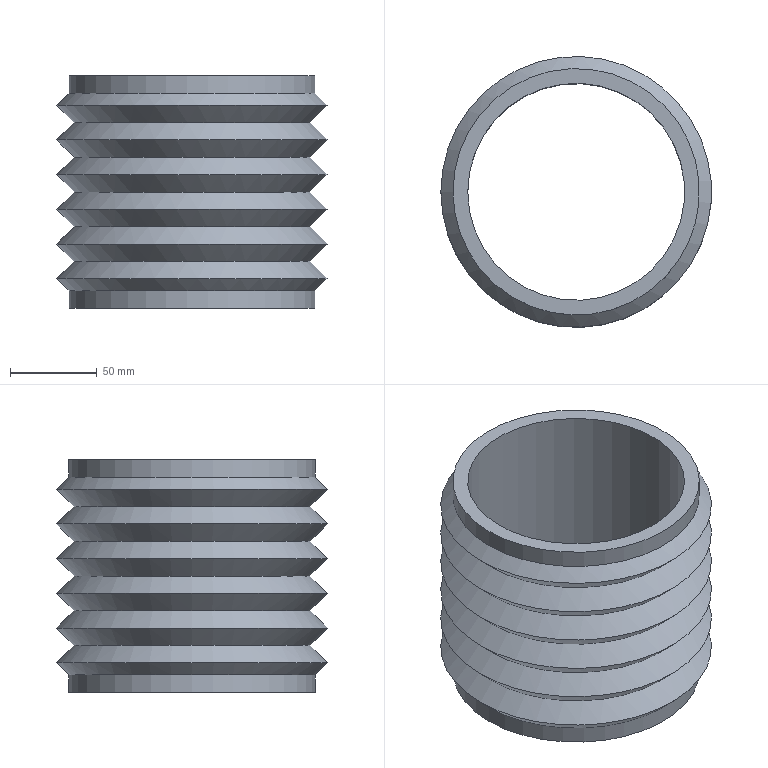Component | NX | CH3404_9-2 | 1 solid | 17 faces | box 156 x 156 x 134 mm | volume 593373 mm3 | cone 12 | cylinder 3 | plane 2 | commonest cylinder face diameters 142 x2 125 x1
STEP:
#1=CARTESIAN_POINT('',(0.,0.,0.));
#2=DIRECTION('',(0.,0.,1.));
#3=DIRECTION('',(1.,0.,0.));
#4=AXIS2_PLACEMENT_3D('',#1,#2,#3);
#5=CARTESIAN_POINT('',(-62.5,0.,0.));
#6=VERTEX_POINT('',#5);
#7=CARTESIAN_POINT('',(0.,0.,0.));
#8=DIRECTION('',(0.,0.,-1.));
#9=DIRECTION('',(-1.,0.,0.));
#10=AXIS2_PLACEMENT_3D('',#7,#8,#9);
#11=CIRCLE('',#10,62.5);
#12=CARTESIAN_POINT('',(0.,0.,-134.));
#13=DIRECTION('',(0.,0.,-1.));
#14=DIRECTION('',(-1.,0.,0.));
#15=AXIS2_PLACEMENT_3D('',#12,#13,#14);
#16=CYLINDRICAL_SURFACE('',#15,62.5);
#17=CARTESIAN_POINT('',(0.,-134.));
#18=DIRECTION('',(1.,0.));
#19=VECTOR('',#18,1.);
#20=LINE('',#17,#19);
#21=(GEOMETRIC_REPRESENTATION_CONTEXT(2)PARAMETRIC_REPRESENTATION_CONTEXT()REPRESENTATION_CONTEXT('',''));
#22=DEFINITIONAL_REPRESENTATION('',(#20),#21);
#23=PCURVE('',#16,#22);
#24=CARTESIAN_POINT('',(-62.5,0.,0.));
#25=DIRECTION('',(0.,0.,-1.));
#26=DIRECTION('',(-1.,0.,0.));
#27=AXIS2_PLACEMENT_3D('',#24,#25,#26);
#28=PLANE('',#27);
#29=CARTESIAN_POINT('',(-62.5,0.));
#30=DIRECTION('',(1.,0.));
#31=AXIS2_PLACEMENT_2D('',#29,#30);
#32=CIRCLE('',#31,62.5);
#33=(GEOMETRIC_REPRESENTATION_CONTEXT(2)PARAMETRIC_REPRESENTATION_CONTEXT()REPRESENTATION_CONTEXT('',''));
#34=DEFINITIONAL_REPRESENTATION('',(#32),#33);
#35=PCURVE('',#28,#34);
#36=SURFACE_CURVE('',#11,(#23,#35),.PCURVE_S1.);
#37=EDGE_CURVE('',#6,#6,#36,.T.);
#38=ORIENTED_EDGE('',*,*,#37,.T.);
#39=CARTESIAN_POINT('',(-62.5,0.,-134.));
#40=VERTEX_POINT('',#39);
#41=CARTESIAN_POINT('',(-62.5,0.,0.));
#42=CARTESIAN_POINT('',(-62.5,0.,-134.));
#43=B_SPLINE_CURVE_WITH_KNOTS('',1,(#41,#42),.UNSPECIFIED.,.F.,.F.,(2,2),(-134.,0.),.PIECEWISE_BEZIER_KNOTS.);
#44=CARTESIAN_POINT('',(6.283,0.));
#45=DIRECTION('',(0.,1.));
#46=VECTOR('',#45,1.);
#47=LINE('',#44,#46);
#48=(GEOMETRIC_REPRESENTATION_CONTEXT(2)PARAMETRIC_REPRESENTATION_CONTEXT()REPRESENTATION_CONTEXT('',''));
#49=DEFINITIONAL_REPRESENTATION('',(#47),#48);
#50=PCURVE('',#16,#49);
#51=CARTESIAN_POINT('',(0.,0.));
#52=DIRECTION('',(0.,1.));
#53=VECTOR('',#52,1.);
#54=LINE('',#51,#53);
#55=(GEOMETRIC_REPRESENTATION_CONTEXT(2)PARAMETRIC_REPRESENTATION_CONTEXT()REPRESENTATION_CONTEXT('',''));
#56=DEFINITIONAL_REPRESENTATION('',(#54),#55);
#57=PCURVE('',#16,#56);
#58=SEAM_CURVE('',#43,(#50,#57),.PCURVE_S1.);
#59=EDGE_CURVE('',#6,#40,#58,.T.);
#60=ORIENTED_EDGE('',*,*,#59,.T.);
#61=CARTESIAN_POINT('',(0.,0.,-134.));
#62=DIRECTION('',(0.,0.,-1.));
#63=DIRECTION('',(-1.,0.,0.));
#64=AXIS2_PLACEMENT_3D('',#61,#62,#63);
#65=CIRCLE('',#64,62.5);
#66=CARTESIAN_POINT('',(0.,0.));
#67=DIRECTION('',(1.,0.));
#68=VECTOR('',#67,1.);
#69=LINE('',#66,#68);
#70=(GEOMETRIC_REPRESENTATION_CONTEXT(2)PARAMETRIC_REPRESENTATION_CONTEXT()REPRESENTATION_CONTEXT('',''));
#71=DEFINITIONAL_REPRESENTATION('',(#69),#70);
#72=PCURVE('',#16,#71);
#73=CARTESIAN_POINT('',(-71.,0.,-134.));
#74=DIRECTION('',(0.,0.,1.));
#75=DIRECTION('',(1.,0.,0.));
#76=AXIS2_PLACEMENT_3D('',#73,#74,#75);
#77=PLANE('',#76);
#78=CARTESIAN_POINT('',(8.5,0.));
#79=CARTESIAN_POINT('',(8.5,108.253));
#80=CARTESIAN_POINT('',(102.25,54.127));
#81=CARTESIAN_POINT('',(196.,0.));
#82=CARTESIAN_POINT('',(102.25,-54.127));
#83=CARTESIAN_POINT('',(8.5,-108.253));
#84=CARTESIAN_POINT('',(8.5,0.));
#85=(BOUNDED_CURVE()B_SPLINE_CURVE(2,(#78,#79,#80,#81,#82,#83,#84),.UNSPECIFIED.,.T.,.F.)B_SPLINE_CURVE_WITH_KNOTS((1,2,2,2,2,1),(-2.094,0.,2.094,4.189,6.283,8.378),.UNSPECIFIED.)CURVE()GEOMETRIC_REPRESENTATION_ITEM()RATIONAL_B_SPLINE_CURVE((1.,0.5,1.,0.5,1.,0.5,1.))REPRESENTATION_ITEM(''));
#86=(GEOMETRIC_REPRESENTATION_CONTEXT(2)PARAMETRIC_REPRESENTATION_CONTEXT()REPRESENTATION_CONTEXT('',''));
#87=DEFINITIONAL_REPRESENTATION('',(#85),#86);
#88=PCURVE('',#77,#87);
#89=SURFACE_CURVE('',#65,(#72,#88),.PCURVE_S1.);
#90=EDGE_CURVE('',#40,#40,#89,.T.);
#91=ORIENTED_EDGE('',*,*,#90,.F.);
#92=ORIENTED_EDGE('',*,*,#59,.F.);
#93=EDGE_LOOP('',(#38,#60,#91,#92));
#94=FACE_BOUND('',#93,.F.);
#95=ADVANCED_FACE('',(#94),#16,.F.);
#96=CARTESIAN_POINT('',(-71.,0.,-0.));
#97=VERTEX_POINT('',#96);
#98=CARTESIAN_POINT('',(0.,0.,-0.));
#99=DIRECTION('',(0.,0.,-1.));
#100=DIRECTION('',(-1.,0.,0.));
#101=AXIS2_PLACEMENT_3D('',#98,#99,#100);
#102=CIRCLE('',#101,71.);
#103=CARTESIAN_POINT('',(-62.5,0.));
#104=DIRECTION('',(1.,0.));
#105=AXIS2_PLACEMENT_2D('',#103,#104);
#106=CIRCLE('',#105,71.);
#107=(GEOMETRIC_REPRESENTATION_CONTEXT(2)PARAMETRIC_REPRESENTATION_CONTEXT()REPRESENTATION_CONTEXT('',''));
#108=DEFINITIONAL_REPRESENTATION('',(#106),#107);
#109=PCURVE('',#28,#108);
#110=CARTESIAN_POINT('',(0.,0.,-134.));
#111=DIRECTION('',(0.,0.,-1.));
#112=DIRECTION('',(-1.,0.,0.));
#113=AXIS2_PLACEMENT_3D('',#110,#111,#112);
#114=CYLINDRICAL_SURFACE('',#113,71.);
#115=CARTESIAN_POINT('',(0.,-134.));
#116=DIRECTION('',(1.,0.));
#117=VECTOR('',#116,1.);
#118=LINE('',#115,#117);
#119=(GEOMETRIC_REPRESENTATION_CONTEXT(2)PARAMETRIC_REPRESENTATION_CONTEXT()REPRESENTATION_CONTEXT('',''));
#120=DEFINITIONAL_REPRESENTATION('',(#118),#119);
#121=PCURVE('',#114,#120);
#122=SURFACE_CURVE('',#102,(#109,#121),.PCURVE_S1.);
#123=EDGE_CURVE('',#97,#97,#122,.T.);
#124=ORIENTED_EDGE('',*,*,#123,.F.);
#125=EDGE_LOOP('',(#124));
#126=FACE_BOUND('',#125,.T.);
#127=ORIENTED_EDGE('',*,*,#37,.T.);
#128=EDGE_LOOP('',(#127));
#129=FACE_BOUND('',#128,.T.);
#130=ADVANCED_FACE('',(#126,#129),#28,.F.);
#131=CARTESIAN_POINT('',(-71.,0.,-10.));
#132=VERTEX_POINT('',#131);
#133=CARTESIAN_POINT('',(0.,0.,-10.));
#134=DIRECTION('',(0.,0.,-1.));
#135=DIRECTION('',(-1.,0.,0.));
#136=AXIS2_PLACEMENT_3D('',#133,#134,#135);
#137=CIRCLE('',#136,71.);
#138=CARTESIAN_POINT('',(0.,-124.));
#139=DIRECTION('',(1.,0.));
#140=VECTOR('',#139,1.);
#141=LINE('',#138,#140);
#142=(GEOMETRIC_REPRESENTATION_CONTEXT(2)PARAMETRIC_REPRESENTATION_CONTEXT()REPRESENTATION_CONTEXT('',''));
#143=DEFINITIONAL_REPRESENTATION('',(#141),#142);
#144=PCURVE('',#114,#143);
#145=CARTESIAN_POINT('',(0.,0.,-10.));
#146=DIRECTION('',(0.,0.,-1.));
#147=DIRECTION('',(-1.,0.,0.));
#148=AXIS2_PLACEMENT_3D('',#145,#146,#147);
#149=CONICAL_SURFACE('',#148,71.,0.7854);
#150=CARTESIAN_POINT('',(0.,0.));
#151=DIRECTION('',(1.,0.));
#152=VECTOR('',#151,1.);
#153=LINE('',#150,#152);
#154=(GEOMETRIC_REPRESENTATION_CONTEXT(2)PARAMETRIC_REPRESENTATION_CONTEXT()REPRESENTATION_CONTEXT('',''));
#155=DEFINITIONAL_REPRESENTATION('',(#153),#154);
#156=PCURVE('',#149,#155);
#157=SURFACE_CURVE('',#137,(#144,#156),.PCURVE_S1.);
#158=EDGE_CURVE('',#132,#132,#157,.T.);
#159=ORIENTED_EDGE('',*,*,#158,.F.);
#160=CARTESIAN_POINT('',(-71.,-0.,-0.));
#161=CARTESIAN_POINT('',(-71.,-0.,-10.));
#162=B_SPLINE_CURVE_WITH_KNOTS('',1,(#160,#161),.UNSPECIFIED.,.F.,.F.,(2,2),(-134.,-124.),.PIECEWISE_BEZIER_KNOTS.);
#163=CARTESIAN_POINT('',(0.,0.));
#164=DIRECTION('',(0.,1.));
#165=VECTOR('',#164,1.);
#166=LINE('',#163,#165);
#167=(GEOMETRIC_REPRESENTATION_CONTEXT(2)PARAMETRIC_REPRESENTATION_CONTEXT()REPRESENTATION_CONTEXT('',''));
#168=DEFINITIONAL_REPRESENTATION('',(#166),#167);
#169=PCURVE('',#114,#168);
#170=CARTESIAN_POINT('',(6.283,0.));
#171=DIRECTION('',(0.,1.));
#172=VECTOR('',#171,1.);
#173=LINE('',#170,#172);
#174=(GEOMETRIC_REPRESENTATION_CONTEXT(2)PARAMETRIC_REPRESENTATION_CONTEXT()REPRESENTATION_CONTEXT('',''));
#175=DEFINITIONAL_REPRESENTATION('',(#173),#174);
#176=PCURVE('',#114,#175);
#177=SEAM_CURVE('',#162,(#169,#176),.PCURVE_S1.);
#178=EDGE_CURVE('',#97,#132,#177,.T.);
#179=ORIENTED_EDGE('',*,*,#178,.F.);
#180=ORIENTED_EDGE('',*,*,#123,.T.);
#181=ORIENTED_EDGE('',*,*,#178,.T.);
#182=EDGE_LOOP('',(#159,#179,#180,#181));
#183=FACE_BOUND('',#182,.T.);
#184=ADVANCED_FACE('',(#183),#114,.T.);
#185=CARTESIAN_POINT('',(-78.,0.,-17.));
#186=VERTEX_POINT('',#185);
#187=CARTESIAN_POINT('',(0.,0.,-17.));
#188=DIRECTION('',(0.,0.,-1.));
#189=DIRECTION('',(-1.,0.,0.));
#190=AXIS2_PLACEMENT_3D('',#187,#188,#189);
#191=CIRCLE('',#190,78.);
#192=CARTESIAN_POINT('',(0.,7.));
#193=DIRECTION('',(1.,0.));
#194=VECTOR('',#193,1.);
#195=LINE('',#192,#194);
#196=(GEOMETRIC_REPRESENTATION_CONTEXT(2)PARAMETRIC_REPRESENTATION_CONTEXT()REPRESENTATION_CONTEXT('',''));
#197=DEFINITIONAL_REPRESENTATION('',(#195),#196);
#198=PCURVE('',#149,#197);
#199=CARTESIAN_POINT('',(0.,0.,-17.));
#200=DIRECTION('',(0.,0.,1.));
#201=DIRECTION('',(1.,0.,0.));
#202=AXIS2_PLACEMENT_3D('',#199,#200,#201);
#203=CONICAL_SURFACE('',#202,78.,0.7854);
#204=CARTESIAN_POINT('',(9.425,0.));
#205=DIRECTION('',(-1.,0.));
#206=VECTOR('',#205,1.);
#207=LINE('',#204,#206);
#208=(GEOMETRIC_REPRESENTATION_CONTEXT(2)PARAMETRIC_REPRESENTATION_CONTEXT()REPRESENTATION_CONTEXT('',''));
#209=DEFINITIONAL_REPRESENTATION('',(#207),#208);
#210=PCURVE('',#203,#209);
#211=SURFACE_CURVE('',#191,(#198,#210),.PCURVE_S1.);
#212=EDGE_CURVE('',#186,#186,#211,.T.);
#213=ORIENTED_EDGE('',*,*,#212,.F.);
#214=CARTESIAN_POINT('',(-71.,-0.,-10.));
#215=CARTESIAN_POINT('',(-78.,-0.,-17.));
#216=B_SPLINE_CURVE_WITH_KNOTS('',1,(#214,#215),.UNSPECIFIED.,.F.,.F.,(2,2),(0.,9.899),.PIECEWISE_BEZIER_KNOTS.);
#217=CARTESIAN_POINT('',(0.,0.));
#218=DIRECTION('',(0.,1.));
#219=VECTOR('',#218,1.);
#220=LINE('',#217,#219);
#221=(GEOMETRIC_REPRESENTATION_CONTEXT(2)PARAMETRIC_REPRESENTATION_CONTEXT()REPRESENTATION_CONTEXT('',''));
#222=DEFINITIONAL_REPRESENTATION('',(#220),#221);
#223=PCURVE('',#149,#222);
#224=CARTESIAN_POINT('',(6.283,0.));
#225=DIRECTION('',(0.,1.));
#226=VECTOR('',#225,1.);
#227=LINE('',#224,#226);
#228=(GEOMETRIC_REPRESENTATION_CONTEXT(2)PARAMETRIC_REPRESENTATION_CONTEXT()REPRESENTATION_CONTEXT('',''));
#229=DEFINITIONAL_REPRESENTATION('',(#227),#228);
#230=PCURVE('',#149,#229);
#231=SEAM_CURVE('',#216,(#223,#230),.PCURVE_S1.);
#232=EDGE_CURVE('',#132,#186,#231,.T.);
#233=ORIENTED_EDGE('',*,*,#232,.F.);
#234=ORIENTED_EDGE('',*,*,#158,.T.);
#235=ORIENTED_EDGE('',*,*,#232,.T.);
#236=EDGE_LOOP('',(#213,#233,#234,#235));
#237=FACE_BOUND('',#236,.T.);
#238=ADVANCED_FACE('',(#237),#149,.T.);
#239=CARTESIAN_POINT('',(-68.,0.,-27.));
#240=VERTEX_POINT('',#239);
#241=CARTESIAN_POINT('',(0.,0.,-27.));
#242=DIRECTION('',(0.,0.,-1.));
#243=DIRECTION('',(-1.,0.,0.));
#244=AXIS2_PLACEMENT_3D('',#241,#242,#243);
#245=CIRCLE('',#244,68.);
#246=CARTESIAN_POINT('',(9.425,-10.));
#247=DIRECTION('',(-1.,0.));
#248=VECTOR('',#247,1.);
#249=LINE('',#246,#248);
#250=(GEOMETRIC_REPRESENTATION_CONTEXT(2)PARAMETRIC_REPRESENTATION_CONTEXT()REPRESENTATION_CONTEXT('',''));
#251=DEFINITIONAL_REPRESENTATION('',(#249),#250);
#252=PCURVE('',#203,#251);
#253=CARTESIAN_POINT('',(0.,0.,-27.));
#254=DIRECTION('',(0.,0.,-1.));
#255=DIRECTION('',(-1.,0.,0.));
#256=AXIS2_PLACEMENT_3D('',#253,#254,#255);
#257=CONICAL_SURFACE('',#256,68.,0.7854);
#258=CARTESIAN_POINT('',(0.,0.));
#259=DIRECTION('',(1.,0.));
#260=VECTOR('',#259,1.);
#261=LINE('',#258,#260);
#262=(GEOMETRIC_REPRESENTATION_CONTEXT(2)PARAMETRIC_REPRESENTATION_CONTEXT()REPRESENTATION_CONTEXT('',''));
#263=DEFINITIONAL_REPRESENTATION('',(#261),#262);
#264=PCURVE('',#257,#263);
#265=SURFACE_CURVE('',#245,(#252,#264),.PCURVE_S1.);
#266=EDGE_CURVE('',#240,#240,#265,.T.);
#267=ORIENTED_EDGE('',*,*,#266,.F.);
#268=CARTESIAN_POINT('',(-68.,0.,-27.));
#269=CARTESIAN_POINT('',(-78.,0.,-17.));
#270=B_SPLINE_CURVE_WITH_KNOTS('',1,(#268,#269),.UNSPECIFIED.,.F.,.F.,(2,2),(-14.142,0.),.PIECEWISE_BEZIER_KNOTS.);
#271=CARTESIAN_POINT('',(9.425,0.));
#272=DIRECTION('',(0.,1.));
#273=VECTOR('',#272,1.);
#274=LINE('',#271,#273);
#275=(GEOMETRIC_REPRESENTATION_CONTEXT(2)PARAMETRIC_REPRESENTATION_CONTEXT()REPRESENTATION_CONTEXT('',''));
#276=DEFINITIONAL_REPRESENTATION('',(#274),#275);
#277=PCURVE('',#203,#276);
#278=CARTESIAN_POINT('',(3.142,0.));
#279=DIRECTION('',(0.,1.));
#280=VECTOR('',#279,1.);
#281=LINE('',#278,#280);
#282=(GEOMETRIC_REPRESENTATION_CONTEXT(2)PARAMETRIC_REPRESENTATION_CONTEXT()REPRESENTATION_CONTEXT('',''));
#283=DEFINITIONAL_REPRESENTATION('',(#281),#282);
#284=PCURVE('',#203,#283);
#285=SEAM_CURVE('',#270,(#277,#284),.PCURVE_S1.);
#286=EDGE_CURVE('',#240,#186,#285,.T.);
#287=ORIENTED_EDGE('',*,*,#286,.T.);
#288=ORIENTED_EDGE('',*,*,#212,.T.);
#289=ORIENTED_EDGE('',*,*,#286,.F.);
#290=EDGE_LOOP('',(#267,#287,#288,#289));
#291=FACE_BOUND('',#290,.T.);
#292=ADVANCED_FACE('',(#291),#203,.T.);
#293=CARTESIAN_POINT('',(-78.,0.,-37.));
#294=VERTEX_POINT('',#293);
#295=CARTESIAN_POINT('',(0.,0.,-37.));
#296=DIRECTION('',(0.,0.,-1.));
#297=DIRECTION('',(-1.,0.,0.));
#298=AXIS2_PLACEMENT_3D('',#295,#296,#297);
#299=CIRCLE('',#298,78.);
#300=CARTESIAN_POINT('',(0.,10.));
#301=DIRECTION('',(1.,0.));
#302=VECTOR('',#301,1.);
#303=LINE('',#300,#302);
#304=(GEOMETRIC_REPRESENTATION_CONTEXT(2)PARAMETRIC_REPRESENTATION_CONTEXT()REPRESENTATION_CONTEXT('',''));
#305=DEFINITIONAL_REPRESENTATION('',(#303),#304);
#306=PCURVE('',#257,#305);
#307=CARTESIAN_POINT('',(0.,0.,-37.));
#308=DIRECTION('',(0.,0.,1.));
#309=DIRECTION('',(1.,0.,0.));
#310=AXIS2_PLACEMENT_3D('',#307,#308,#309);
#311=CONICAL_SURFACE('',#310,78.,0.7854);
#312=CARTESIAN_POINT('',(9.425,0.));
#313=DIRECTION('',(-1.,0.));
#314=VECTOR('',#313,1.);
#315=LINE('',#312,#314);
#316=(GEOMETRIC_REPRESENTATION_CONTEXT(2)PARAMETRIC_REPRESENTATION_CONTEXT()REPRESENTATION_CONTEXT('',''));
#317=DEFINITIONAL_REPRESENTATION('',(#315),#316);
#318=PCURVE('',#311,#317);
#319=SURFACE_CURVE('',#299,(#306,#318),.PCURVE_S1.);
#320=EDGE_CURVE('',#294,#294,#319,.T.);
#321=ORIENTED_EDGE('',*,*,#320,.F.);
#322=CARTESIAN_POINT('',(-68.,-0.,-27.));
#323=CARTESIAN_POINT('',(-78.,-0.,-37.));
#324=B_SPLINE_CURVE_WITH_KNOTS('',1,(#322,#323),.UNSPECIFIED.,.F.,.F.,(2,2),(0.,14.142),.PIECEWISE_BEZIER_KNOTS.);
#325=CARTESIAN_POINT('',(0.,0.));
#326=DIRECTION('',(0.,1.));
#327=VECTOR('',#326,1.);
#328=LINE('',#325,#327);
#329=(GEOMETRIC_REPRESENTATION_CONTEXT(2)PARAMETRIC_REPRESENTATION_CONTEXT()REPRESENTATION_CONTEXT('',''));
#330=DEFINITIONAL_REPRESENTATION('',(#328),#329);
#331=PCURVE('',#257,#330);
#332=CARTESIAN_POINT('',(6.283,0.));
#333=DIRECTION('',(0.,1.));
#334=VECTOR('',#333,1.);
#335=LINE('',#332,#334);
#336=(GEOMETRIC_REPRESENTATION_CONTEXT(2)PARAMETRIC_REPRESENTATION_CONTEXT()REPRESENTATION_CONTEXT('',''));
#337=DEFINITIONAL_REPRESENTATION('',(#335),#336);
#338=PCURVE('',#257,#337);
#339=SEAM_CURVE('',#324,(#331,#338),.PCURVE_S1.);
#340=EDGE_CURVE('',#240,#294,#339,.T.);
#341=ORIENTED_EDGE('',*,*,#340,.F.);
#342=ORIENTED_EDGE('',*,*,#266,.T.);
#343=ORIENTED_EDGE('',*,*,#340,.T.);
#344=EDGE_LOOP('',(#321,#341,#342,#343));
#345=FACE_BOUND('',#344,.T.);
#346=ADVANCED_FACE('',(#345),#257,.T.);
#347=CARTESIAN_POINT('',(-68.,0.,-47.));
#348=VERTEX_POINT('',#347);
#349=CARTESIAN_POINT('',(0.,0.,-47.));
#350=DIRECTION('',(0.,0.,-1.));
#351=DIRECTION('',(-1.,0.,0.));
#352=AXIS2_PLACEMENT_3D('',#349,#350,#351);
#353=CIRCLE('',#352,68.);
#354=CARTESIAN_POINT('',(9.425,-10.));
#355=DIRECTION('',(-1.,0.));
#356=VECTOR('',#355,1.);
#357=LINE('',#354,#356);
#358=(GEOMETRIC_REPRESENTATION_CONTEXT(2)PARAMETRIC_REPRESENTATION_CONTEXT()REPRESENTATION_CONTEXT('',''));
#359=DEFINITIONAL_REPRESENTATION('',(#357),#358);
#360=PCURVE('',#311,#359);
#361=CARTESIAN_POINT('',(0.,0.,-47.));
#362=DIRECTION('',(0.,0.,-1.));
#363=DIRECTION('',(-1.,0.,0.));
#364=AXIS2_PLACEMENT_3D('',#361,#362,#363);
#365=CONICAL_SURFACE('',#364,68.,0.7854);
#366=CARTESIAN_POINT('',(0.,0.));
#367=DIRECTION('',(1.,0.));
#368=VECTOR('',#367,1.);
#369=LINE('',#366,#368);
#370=(GEOMETRIC_REPRESENTATION_CONTEXT(2)PARAMETRIC_REPRESENTATION_CONTEXT()REPRESENTATION_CONTEXT('',''));
#371=DEFINITIONAL_REPRESENTATION('',(#369),#370);
#372=PCURVE('',#365,#371);
#373=SURFACE_CURVE('',#353,(#360,#372),.PCURVE_S1.);
#374=EDGE_CURVE('',#348,#348,#373,.T.);
#375=ORIENTED_EDGE('',*,*,#374,.F.);
#376=CARTESIAN_POINT('',(-68.,0.,-47.));
#377=CARTESIAN_POINT('',(-78.,0.,-37.));
#378=B_SPLINE_CURVE_WITH_KNOTS('',1,(#376,#377),.UNSPECIFIED.,.F.,.F.,(2,2),(-14.142,0.),.PIECEWISE_BEZIER_KNOTS.);
#379=CARTESIAN_POINT('',(9.425,0.));
#380=DIRECTION('',(0.,1.));
#381=VECTOR('',#380,1.);
#382=LINE('',#379,#381);
#383=(GEOMETRIC_REPRESENTATION_CONTEXT(2)PARAMETRIC_REPRESENTATION_CONTEXT()REPRESENTATION_CONTEXT('',''));
#384=DEFINITIONAL_REPRESENTATION('',(#382),#383);
#385=PCURVE('',#311,#384);
#386=CARTESIAN_POINT('',(3.142,0.));
#387=DIRECTION('',(0.,1.));
#388=VECTOR('',#387,1.);
#389=LINE('',#386,#388);
#390=(GEOMETRIC_REPRESENTATION_CONTEXT(2)PARAMETRIC_REPRESENTATION_CONTEXT()REPRESENTATION_CONTEXT('',''));
#391=DEFINITIONAL_REPRESENTATION('',(#389),#390);
#392=PCURVE('',#311,#391);
#393=SEAM_CURVE('',#378,(#385,#392),.PCURVE_S1.);
#394=EDGE_CURVE('',#348,#294,#393,.T.);
#395=ORIENTED_EDGE('',*,*,#394,.T.);
#396=ORIENTED_EDGE('',*,*,#320,.T.);
#397=ORIENTED_EDGE('',*,*,#394,.F.);
#398=EDGE_LOOP('',(#375,#395,#396,#397));
#399=FACE_BOUND('',#398,.T.);
#400=ADVANCED_FACE('',(#399),#311,.T.);
#401=CARTESIAN_POINT('',(-78.,0.,-57.));
#402=VERTEX_POINT('',#401);
#403=CARTESIAN_POINT('',(0.,0.,-57.));
#404=DIRECTION('',(0.,0.,-1.));
#405=DIRECTION('',(-1.,0.,0.));
#406=AXIS2_PLACEMENT_3D('',#403,#404,#405);
#407=CIRCLE('',#406,78.);
#408=CARTESIAN_POINT('',(0.,10.));
#409=DIRECTION('',(1.,0.));
#410=VECTOR('',#409,1.);
#411=LINE('',#408,#410);
#412=(GEOMETRIC_REPRESENTATION_CONTEXT(2)PARAMETRIC_REPRESENTATION_CONTEXT()REPRESENTATION_CONTEXT('',''));
#413=DEFINITIONAL_REPRESENTATION('',(#411),#412);
#414=PCURVE('',#365,#413);
#415=CARTESIAN_POINT('',(0.,0.,-57.));
#416=DIRECTION('',(0.,0.,1.));
#417=DIRECTION('',(1.,0.,0.));
#418=AXIS2_PLACEMENT_3D('',#415,#416,#417);
#419=CONICAL_SURFACE('',#418,78.,0.7854);
#420=CARTESIAN_POINT('',(9.425,0.));
#421=DIRECTION('',(-1.,0.));
#422=VECTOR('',#421,1.);
#423=LINE('',#420,#422);
#424=(GEOMETRIC_REPRESENTATION_CONTEXT(2)PARAMETRIC_REPRESENTATION_CONTEXT()REPRESENTATION_CONTEXT('',''));
#425=DEFINITIONAL_REPRESENTATION('',(#423),#424);
#426=PCURVE('',#419,#425);
#427=SURFACE_CURVE('',#407,(#414,#426),.PCURVE_S1.);
#428=EDGE_CURVE('',#402,#402,#427,.T.);
#429=ORIENTED_EDGE('',*,*,#428,.F.);
#430=CARTESIAN_POINT('',(-68.,-0.,-47.));
#431=CARTESIAN_POINT('',(-78.,-0.,-57.));
#432=B_SPLINE_CURVE_WITH_KNOTS('',1,(#430,#431),.UNSPECIFIED.,.F.,.F.,(2,2),(0.,14.142),.PIECEWISE_BEZIER_KNOTS.);
#433=CARTESIAN_POINT('',(0.,0.));
#434=DIRECTION('',(0.,1.));
#435=VECTOR('',#434,1.);
#436=LINE('',#433,#435);
#437=(GEOMETRIC_REPRESENTATION_CONTEXT(2)PARAMETRIC_REPRESENTATION_CONTEXT()REPRESENTATION_CONTEXT('',''));
#438=DEFINITIONAL_REPRESENTATION('',(#436),#437);
#439=PCURVE('',#365,#438);
#440=CARTESIAN_POINT('',(6.283,0.));
#441=DIRECTION('',(0.,1.));
#442=VECTOR('',#441,1.);
#443=LINE('',#440,#442);
#444=(GEOMETRIC_REPRESENTATION_CONTEXT(2)PARAMETRIC_REPRESENTATION_CONTEXT()REPRESENTATION_CONTEXT('',''));
#445=DEFINITIONAL_REPRESENTATION('',(#443),#444);
#446=PCURVE('',#365,#445);
#447=SEAM_CURVE('',#432,(#439,#446),.PCURVE_S1.);
#448=EDGE_CURVE('',#348,#402,#447,.T.);
#449=ORIENTED_EDGE('',*,*,#448,.F.);
#450=ORIENTED_EDGE('',*,*,#374,.T.);
#451=ORIENTED_EDGE('',*,*,#448,.T.);
#452=EDGE_LOOP('',(#429,#449,#450,#451));
#453=FACE_BOUND('',#452,.T.);
#454=ADVANCED_FACE('',(#453),#365,.T.);
#455=CARTESIAN_POINT('',(-68.,0.,-67.));
#456=VERTEX_POINT('',#455);
#457=CARTESIAN_POINT('',(0.,0.,-67.));
#458=DIRECTION('',(0.,0.,-1.));
#459=DIRECTION('',(-1.,0.,0.));
#460=AXIS2_PLACEMENT_3D('',#457,#458,#459);
#461=CIRCLE('',#460,68.);
#462=CARTESIAN_POINT('',(9.425,-10.));
#463=DIRECTION('',(-1.,0.));
#464=VECTOR('',#463,1.);
#465=LINE('',#462,#464);
#466=(GEOMETRIC_REPRESENTATION_CONTEXT(2)PARAMETRIC_REPRESENTATION_CONTEXT()REPRESENTATION_CONTEXT('',''));
#467=DEFINITIONAL_REPRESENTATION('',(#465),#466);
#468=PCURVE('',#419,#467);
#469=CARTESIAN_POINT('',(0.,0.,-67.));
#470=DIRECTION('',(0.,0.,-1.));
#471=DIRECTION('',(-1.,0.,0.));
#472=AXIS2_PLACEMENT_3D('',#469,#470,#471);
#473=CONICAL_SURFACE('',#472,68.,0.7854);
#474=CARTESIAN_POINT('',(0.,0.));
#475=DIRECTION('',(1.,0.));
#476=VECTOR('',#475,1.);
#477=LINE('',#474,#476);
#478=(GEOMETRIC_REPRESENTATION_CONTEXT(2)PARAMETRIC_REPRESENTATION_CONTEXT()REPRESENTATION_CONTEXT('',''));
#479=DEFINITIONAL_REPRESENTATION('',(#477),#478);
#480=PCURVE('',#473,#479);
#481=SURFACE_CURVE('',#461,(#468,#480),.PCURVE_S1.);
#482=EDGE_CURVE('',#456,#456,#481,.T.);
#483=ORIENTED_EDGE('',*,*,#482,.F.);
#484=CARTESIAN_POINT('',(-68.,0.,-67.));
#485=CARTESIAN_POINT('',(-78.,0.,-57.));
#486=B_SPLINE_CURVE_WITH_KNOTS('',1,(#484,#485),.UNSPECIFIED.,.F.,.F.,(2,2),(-14.142,0.),.PIECEWISE_BEZIER_KNOTS.);
#487=CARTESIAN_POINT('',(9.425,0.));
#488=DIRECTION('',(0.,1.));
#489=VECTOR('',#488,1.);
#490=LINE('',#487,#489);
#491=(GEOMETRIC_REPRESENTATION_CONTEXT(2)PARAMETRIC_REPRESENTATION_CONTEXT()REPRESENTATION_CONTEXT('',''));
#492=DEFINITIONAL_REPRESENTATION('',(#490),#491);
#493=PCURVE('',#419,#492);
#494=CARTESIAN_POINT('',(3.142,0.));
#495=DIRECTION('',(0.,1.));
#496=VECTOR('',#495,1.);
#497=LINE('',#494,#496);
#498=(GEOMETRIC_REPRESENTATION_CONTEXT(2)PARAMETRIC_REPRESENTATION_CONTEXT()REPRESENTATION_CONTEXT('',''));
#499=DEFINITIONAL_REPRESENTATION('',(#497),#498);
#500=PCURVE('',#419,#499);
#501=SEAM_CURVE('',#486,(#493,#500),.PCURVE_S1.);
#502=EDGE_CURVE('',#456,#402,#501,.T.);
#503=ORIENTED_EDGE('',*,*,#502,.T.);
#504=ORIENTED_EDGE('',*,*,#428,.T.);
#505=ORIENTED_EDGE('',*,*,#502,.F.);
#506=EDGE_LOOP('',(#483,#503,#504,#505));
#507=FACE_BOUND('',#506,.T.);
#508=ADVANCED_FACE('',(#507),#419,.T.);
#509=CARTESIAN_POINT('',(-78.,0.,-77.));
#510=VERTEX_POINT('',#509);
#511=CARTESIAN_POINT('',(0.,0.,-77.));
#512=DIRECTION('',(0.,0.,-1.));
#513=DIRECTION('',(-1.,0.,0.));
#514=AXIS2_PLACEMENT_3D('',#511,#512,#513);
#515=CIRCLE('',#514,78.);
#516=CARTESIAN_POINT('',(0.,10.));
#517=DIRECTION('',(1.,0.));
#518=VECTOR('',#517,1.);
#519=LINE('',#516,#518);
#520=(GEOMETRIC_REPRESENTATION_CONTEXT(2)PARAMETRIC_REPRESENTATION_CONTEXT()REPRESENTATION_CONTEXT('',''));
#521=DEFINITIONAL_REPRESENTATION('',(#519),#520);
#522=PCURVE('',#473,#521);
#523=CARTESIAN_POINT('',(0.,0.,-77.));
#524=DIRECTION('',(0.,0.,1.));
#525=DIRECTION('',(1.,0.,0.));
#526=AXIS2_PLACEMENT_3D('',#523,#524,#525);
#527=CONICAL_SURFACE('',#526,78.,0.7854);
#528=CARTESIAN_POINT('',(9.425,0.));
#529=DIRECTION('',(-1.,0.));
#530=VECTOR('',#529,1.);
#531=LINE('',#528,#530);
#532=(GEOMETRIC_REPRESENTATION_CONTEXT(2)PARAMETRIC_REPRESENTATION_CONTEXT()REPRESENTATION_CONTEXT('',''));
#533=DEFINITIONAL_REPRESENTATION('',(#531),#532);
#534=PCURVE('',#527,#533);
#535=SURFACE_CURVE('',#515,(#522,#534),.PCURVE_S1.);
#536=EDGE_CURVE('',#510,#510,#535,.T.);
#537=ORIENTED_EDGE('',*,*,#536,.F.);
#538=CARTESIAN_POINT('',(-68.,-0.,-67.));
#539=CARTESIAN_POINT('',(-78.,-0.,-77.));
#540=B_SPLINE_CURVE_WITH_KNOTS('',1,(#538,#539),.UNSPECIFIED.,.F.,.F.,(2,2),(0.,14.142),.PIECEWISE_BEZIER_KNOTS.);
#541=CARTESIAN_POINT('',(0.,0.));
#542=DIRECTION('',(0.,1.));
#543=VECTOR('',#542,1.);
#544=LINE('',#541,#543);
#545=(GEOMETRIC_REPRESENTATION_CONTEXT(2)PARAMETRIC_REPRESENTATION_CONTEXT()REPRESENTATION_CONTEXT('',''));
#546=DEFINITIONAL_REPRESENTATION('',(#544),#545);
#547=PCURVE('',#473,#546);
#548=CARTESIAN_POINT('',(6.283,0.));
#549=DIRECTION('',(0.,1.));
#550=VECTOR('',#549,1.);
#551=LINE('',#548,#550);
#552=(GEOMETRIC_REPRESENTATION_CONTEXT(2)PARAMETRIC_REPRESENTATION_CONTEXT()REPRESENTATION_CONTEXT('',''));
#553=DEFINITIONAL_REPRESENTATION('',(#551),#552);
#554=PCURVE('',#473,#553);
#555=SEAM_CURVE('',#540,(#547,#554),.PCURVE_S1.);
#556=EDGE_CURVE('',#456,#510,#555,.T.);
#557=ORIENTED_EDGE('',*,*,#556,.F.);
#558=ORIENTED_EDGE('',*,*,#482,.T.);
#559=ORIENTED_EDGE('',*,*,#556,.T.);
#560=EDGE_LOOP('',(#537,#557,#558,#559));
#561=FACE_BOUND('',#560,.T.);
#562=ADVANCED_FACE('',(#561),#473,.T.);
#563=CARTESIAN_POINT('',(-68.,0.,-87.));
#564=VERTEX_POINT('',#563);
#565=CARTESIAN_POINT('',(0.,0.,-87.));
#566=DIRECTION('',(0.,0.,-1.));
#567=DIRECTION('',(-1.,0.,0.));
#568=AXIS2_PLACEMENT_3D('',#565,#566,#567);
#569=CIRCLE('',#568,68.);
#570=CARTESIAN_POINT('',(9.425,-10.));
#571=DIRECTION('',(-1.,0.));
#572=VECTOR('',#571,1.);
#573=LINE('',#570,#572);
#574=(GEOMETRIC_REPRESENTATION_CONTEXT(2)PARAMETRIC_REPRESENTATION_CONTEXT()REPRESENTATION_CONTEXT('',''));
#575=DEFINITIONAL_REPRESENTATION('',(#573),#574);
#576=PCURVE('',#527,#575);
#577=CARTESIAN_POINT('',(0.,0.,-87.));
#578=DIRECTION('',(0.,0.,-1.));
#579=DIRECTION('',(-1.,0.,0.));
#580=AXIS2_PLACEMENT_3D('',#577,#578,#579);
#581=CONICAL_SURFACE('',#580,68.,0.7854);
#582=CARTESIAN_POINT('',(0.,0.));
#583=DIRECTION('',(1.,0.));
#584=VECTOR('',#583,1.);
#585=LINE('',#582,#584);
#586=(GEOMETRIC_REPRESENTATION_CONTEXT(2)PARAMETRIC_REPRESENTATION_CONTEXT()REPRESENTATION_CONTEXT('',''));
#587=DEFINITIONAL_REPRESENTATION('',(#585),#586);
#588=PCURVE('',#581,#587);
#589=SURFACE_CURVE('',#569,(#576,#588),.PCURVE_S1.);
#590=EDGE_CURVE('',#564,#564,#589,.T.);
#591=ORIENTED_EDGE('',*,*,#590,.F.);
#592=CARTESIAN_POINT('',(-68.,0.,-87.));
#593=CARTESIAN_POINT('',(-78.,0.,-77.));
#594=B_SPLINE_CURVE_WITH_KNOTS('',1,(#592,#593),.UNSPECIFIED.,.F.,.F.,(2,2),(-14.142,0.),.PIECEWISE_BEZIER_KNOTS.);
#595=CARTESIAN_POINT('',(9.425,0.));
#596=DIRECTION('',(0.,1.));
#597=VECTOR('',#596,1.);
#598=LINE('',#595,#597);
#599=(GEOMETRIC_REPRESENTATION_CONTEXT(2)PARAMETRIC_REPRESENTATION_CONTEXT()REPRESENTATION_CONTEXT('',''));
#600=DEFINITIONAL_REPRESENTATION('',(#598),#599);
#601=PCURVE('',#527,#600);
#602=CARTESIAN_POINT('',(3.142,0.));
#603=DIRECTION('',(0.,1.));
#604=VECTOR('',#603,1.);
#605=LINE('',#602,#604);
#606=(GEOMETRIC_REPRESENTATION_CONTEXT(2)PARAMETRIC_REPRESENTATION_CONTEXT()REPRESENTATION_CONTEXT('',''));
#607=DEFINITIONAL_REPRESENTATION('',(#605),#606);
#608=PCURVE('',#527,#607);
#609=SEAM_CURVE('',#594,(#601,#608),.PCURVE_S1.);
#610=EDGE_CURVE('',#564,#510,#609,.T.);
#611=ORIENTED_EDGE('',*,*,#610,.T.);
#612=ORIENTED_EDGE('',*,*,#536,.T.);
#613=ORIENTED_EDGE('',*,*,#610,.F.);
#614=EDGE_LOOP('',(#591,#611,#612,#613));
#615=FACE_BOUND('',#614,.T.);
#616=ADVANCED_FACE('',(#615),#527,.T.);
#617=CARTESIAN_POINT('',(-78.,0.,-97.));
#618=VERTEX_POINT('',#617);
#619=CARTESIAN_POINT('',(0.,0.,-97.));
#620=DIRECTION('',(0.,0.,-1.));
#621=DIRECTION('',(-1.,0.,0.));
#622=AXIS2_PLACEMENT_3D('',#619,#620,#621);
#623=CIRCLE('',#622,78.);
#624=CARTESIAN_POINT('',(0.,10.));
#625=DIRECTION('',(1.,0.));
#626=VECTOR('',#625,1.);
#627=LINE('',#624,#626);
#628=(GEOMETRIC_REPRESENTATION_CONTEXT(2)PARAMETRIC_REPRESENTATION_CONTEXT()REPRESENTATION_CONTEXT('',''));
#629=DEFINITIONAL_REPRESENTATION('',(#627),#628);
#630=PCURVE('',#581,#629);
#631=CARTESIAN_POINT('',(0.,0.,-97.));
#632=DIRECTION('',(0.,0.,1.));
#633=DIRECTION('',(1.,0.,0.));
#634=AXIS2_PLACEMENT_3D('',#631,#632,#633);
#635=CONICAL_SURFACE('',#634,78.,0.7854);
#636=CARTESIAN_POINT('',(9.425,0.));
#637=DIRECTION('',(-1.,0.));
#638=VECTOR('',#637,1.);
#639=LINE('',#636,#638);
#640=(GEOMETRIC_REPRESENTATION_CONTEXT(2)PARAMETRIC_REPRESENTATION_CONTEXT()REPRESENTATION_CONTEXT('',''));
#641=DEFINITIONAL_REPRESENTATION('',(#639),#640);
#642=PCURVE('',#635,#641);
#643=SURFACE_CURVE('',#623,(#630,#642),.PCURVE_S1.);
#644=EDGE_CURVE('',#618,#618,#643,.T.);
#645=ORIENTED_EDGE('',*,*,#644,.F.);
#646=CARTESIAN_POINT('',(-68.,-0.,-87.));
#647=CARTESIAN_POINT('',(-78.,-0.,-97.));
#648=B_SPLINE_CURVE_WITH_KNOTS('',1,(#646,#647),.UNSPECIFIED.,.F.,.F.,(2,2),(0.,14.142),.PIECEWISE_BEZIER_KNOTS.);
#649=CARTESIAN_POINT('',(0.,0.));
#650=DIRECTION('',(0.,1.));
#651=VECTOR('',#650,1.);
#652=LINE('',#649,#651);
#653=(GEOMETRIC_REPRESENTATION_CONTEXT(2)PARAMETRIC_REPRESENTATION_CONTEXT()REPRESENTATION_CONTEXT('',''));
#654=DEFINITIONAL_REPRESENTATION('',(#652),#653);
#655=PCURVE('',#581,#654);
#656=CARTESIAN_POINT('',(6.283,0.));
#657=DIRECTION('',(0.,1.));
#658=VECTOR('',#657,1.);
#659=LINE('',#656,#658);
#660=(GEOMETRIC_REPRESENTATION_CONTEXT(2)PARAMETRIC_REPRESENTATION_CONTEXT()REPRESENTATION_CONTEXT('',''));
#661=DEFINITIONAL_REPRESENTATION('',(#659),#660);
#662=PCURVE('',#581,#661);
#663=SEAM_CURVE('',#648,(#655,#662),.PCURVE_S1.);
#664=EDGE_CURVE('',#564,#618,#663,.T.);
#665=ORIENTED_EDGE('',*,*,#664,.F.);
#666=ORIENTED_EDGE('',*,*,#590,.T.);
#667=ORIENTED_EDGE('',*,*,#664,.T.);
#668=EDGE_LOOP('',(#645,#665,#666,#667));
#669=FACE_BOUND('',#668,.T.);
#670=ADVANCED_FACE('',(#669),#581,.T.);
#671=CARTESIAN_POINT('',(-68.,0.,-107.));
#672=VERTEX_POINT('',#671);
#673=CARTESIAN_POINT('',(0.,0.,-107.));
#674=DIRECTION('',(0.,0.,-1.));
#675=DIRECTION('',(-1.,0.,0.));
#676=AXIS2_PLACEMENT_3D('',#673,#674,#675);
#677=CIRCLE('',#676,68.);
#678=CARTESIAN_POINT('',(9.425,-10.));
#679=DIRECTION('',(-1.,0.));
#680=VECTOR('',#679,1.);
#681=LINE('',#678,#680);
#682=(GEOMETRIC_REPRESENTATION_CONTEXT(2)PARAMETRIC_REPRESENTATION_CONTEXT()REPRESENTATION_CONTEXT('',''));
#683=DEFINITIONAL_REPRESENTATION('',(#681),#682);
#684=PCURVE('',#635,#683);
#685=CARTESIAN_POINT('',(0.,0.,-107.));
#686=DIRECTION('',(0.,0.,-1.));
#687=DIRECTION('',(-1.,0.,0.));
#688=AXIS2_PLACEMENT_3D('',#685,#686,#687);
#689=CONICAL_SURFACE('',#688,68.,0.7854);
#690=CARTESIAN_POINT('',(0.,0.));
#691=DIRECTION('',(1.,0.));
#692=VECTOR('',#691,1.);
#693=LINE('',#690,#692);
#694=(GEOMETRIC_REPRESENTATION_CONTEXT(2)PARAMETRIC_REPRESENTATION_CONTEXT()REPRESENTATION_CONTEXT('',''));
#695=DEFINITIONAL_REPRESENTATION('',(#693),#694);
#696=PCURVE('',#689,#695);
#697=SURFACE_CURVE('',#677,(#684,#696),.PCURVE_S1.);
#698=EDGE_CURVE('',#672,#672,#697,.T.);
#699=ORIENTED_EDGE('',*,*,#698,.F.);
#700=CARTESIAN_POINT('',(-68.,0.,-107.));
#701=CARTESIAN_POINT('',(-78.,0.,-97.));
#702=B_SPLINE_CURVE_WITH_KNOTS('',1,(#700,#701),.UNSPECIFIED.,.F.,.F.,(2,2),(-14.142,0.),.PIECEWISE_BEZIER_KNOTS.);
#703=CARTESIAN_POINT('',(9.425,0.));
#704=DIRECTION('',(0.,1.));
#705=VECTOR('',#704,1.);
#706=LINE('',#703,#705);
#707=(GEOMETRIC_REPRESENTATION_CONTEXT(2)PARAMETRIC_REPRESENTATION_CONTEXT()REPRESENTATION_CONTEXT('',''));
#708=DEFINITIONAL_REPRESENTATION('',(#706),#707);
#709=PCURVE('',#635,#708);
#710=CARTESIAN_POINT('',(3.142,0.));
#711=DIRECTION('',(0.,1.));
#712=VECTOR('',#711,1.);
#713=LINE('',#710,#712);
#714=(GEOMETRIC_REPRESENTATION_CONTEXT(2)PARAMETRIC_REPRESENTATION_CONTEXT()REPRESENTATION_CONTEXT('',''));
#715=DEFINITIONAL_REPRESENTATION('',(#713),#714);
#716=PCURVE('',#635,#715);
#717=SEAM_CURVE('',#702,(#709,#716),.PCURVE_S1.);
#718=EDGE_CURVE('',#672,#618,#717,.T.);
#719=ORIENTED_EDGE('',*,*,#718,.T.);
#720=ORIENTED_EDGE('',*,*,#644,.T.);
#721=ORIENTED_EDGE('',*,*,#718,.F.);
#722=EDGE_LOOP('',(#699,#719,#720,#721));
#723=FACE_BOUND('',#722,.T.);
#724=ADVANCED_FACE('',(#723),#635,.T.);
#725=CARTESIAN_POINT('',(-78.,0.,-117.));
#726=VERTEX_POINT('',#725);
#727=CARTESIAN_POINT('',(0.,0.,-117.));
#728=DIRECTION('',(0.,0.,-1.));
#729=DIRECTION('',(-1.,0.,0.));
#730=AXIS2_PLACEMENT_3D('',#727,#728,#729);
#731=CIRCLE('',#730,78.);
#732=CARTESIAN_POINT('',(0.,10.));
#733=DIRECTION('',(1.,0.));
#734=VECTOR('',#733,1.);
#735=LINE('',#732,#734);
#736=(GEOMETRIC_REPRESENTATION_CONTEXT(2)PARAMETRIC_REPRESENTATION_CONTEXT()REPRESENTATION_CONTEXT('',''));
#737=DEFINITIONAL_REPRESENTATION('',(#735),#736);
#738=PCURVE('',#689,#737);
#739=CARTESIAN_POINT('',(0.,0.,-117.));
#740=DIRECTION('',(0.,0.,1.));
#741=DIRECTION('',(1.,0.,0.));
#742=AXIS2_PLACEMENT_3D('',#739,#740,#741);
#743=CONICAL_SURFACE('',#742,78.,0.7854);
#744=CARTESIAN_POINT('',(9.425,0.));
#745=DIRECTION('',(-1.,0.));
#746=VECTOR('',#745,1.);
#747=LINE('',#744,#746);
#748=(GEOMETRIC_REPRESENTATION_CONTEXT(2)PARAMETRIC_REPRESENTATION_CONTEXT()REPRESENTATION_CONTEXT('',''));
#749=DEFINITIONAL_REPRESENTATION('',(#747),#748);
#750=PCURVE('',#743,#749);
#751=SURFACE_CURVE('',#731,(#738,#750),.PCURVE_S1.);
#752=EDGE_CURVE('',#726,#726,#751,.T.);
#753=ORIENTED_EDGE('',*,*,#752,.F.);
#754=CARTESIAN_POINT('',(-68.,-0.,-107.));
#755=CARTESIAN_POINT('',(-78.,-0.,-117.));
#756=B_SPLINE_CURVE_WITH_KNOTS('',1,(#754,#755),.UNSPECIFIED.,.F.,.F.,(2,2),(0.,14.142),.PIECEWISE_BEZIER_KNOTS.);
#757=CARTESIAN_POINT('',(0.,0.));
#758=DIRECTION('',(0.,1.));
#759=VECTOR('',#758,1.);
#760=LINE('',#757,#759);
#761=(GEOMETRIC_REPRESENTATION_CONTEXT(2)PARAMETRIC_REPRESENTATION_CONTEXT()REPRESENTATION_CONTEXT('',''));
#762=DEFINITIONAL_REPRESENTATION('',(#760),#761);
#763=PCURVE('',#689,#762);
#764=CARTESIAN_POINT('',(6.283,0.));
#765=DIRECTION('',(0.,1.));
#766=VECTOR('',#765,1.);
#767=LINE('',#764,#766);
#768=(GEOMETRIC_REPRESENTATION_CONTEXT(2)PARAMETRIC_REPRESENTATION_CONTEXT()REPRESENTATION_CONTEXT('',''));
#769=DEFINITIONAL_REPRESENTATION('',(#767),#768);
#770=PCURVE('',#689,#769);
#771=SEAM_CURVE('',#756,(#763,#770),.PCURVE_S1.);
#772=EDGE_CURVE('',#672,#726,#771,.T.);
#773=ORIENTED_EDGE('',*,*,#772,.F.);
#774=ORIENTED_EDGE('',*,*,#698,.T.);
#775=ORIENTED_EDGE('',*,*,#772,.T.);
#776=EDGE_LOOP('',(#753,#773,#774,#775));
#777=FACE_BOUND('',#776,.T.);
#778=ADVANCED_FACE('',(#777),#689,.T.);
#779=CARTESIAN_POINT('',(-71.,0.,-124.));
#780=VERTEX_POINT('',#779);
#781=CARTESIAN_POINT('',(0.,0.,-124.));
#782=DIRECTION('',(0.,0.,-1.));
#783=DIRECTION('',(-1.,0.,0.));
#784=AXIS2_PLACEMENT_3D('',#781,#782,#783);
#785=CIRCLE('',#784,71.);
#786=CARTESIAN_POINT('',(9.425,-7.));
#787=DIRECTION('',(-1.,0.));
#788=VECTOR('',#787,1.);
#789=LINE('',#786,#788);
#790=(GEOMETRIC_REPRESENTATION_CONTEXT(2)PARAMETRIC_REPRESENTATION_CONTEXT()REPRESENTATION_CONTEXT('',''));
#791=DEFINITIONAL_REPRESENTATION('',(#789),#790);
#792=PCURVE('',#743,#791);
#793=CARTESIAN_POINT('',(0.,0.,-134.));
#794=DIRECTION('',(0.,0.,-1.));
#795=DIRECTION('',(-1.,0.,0.));
#796=AXIS2_PLACEMENT_3D('',#793,#794,#795);
#797=CYLINDRICAL_SURFACE('',#796,71.);
#798=CARTESIAN_POINT('',(0.,-10.));
#799=DIRECTION('',(1.,0.));
#800=VECTOR('',#799,1.);
#801=LINE('',#798,#800);
#802=(GEOMETRIC_REPRESENTATION_CONTEXT(2)PARAMETRIC_REPRESENTATION_CONTEXT()REPRESENTATION_CONTEXT('',''));
#803=DEFINITIONAL_REPRESENTATION('',(#801),#802);
#804=PCURVE('',#797,#803);
#805=SURFACE_CURVE('',#785,(#792,#804),.PCURVE_S1.);
#806=EDGE_CURVE('',#780,#780,#805,.T.);
#807=ORIENTED_EDGE('',*,*,#806,.F.);
#808=CARTESIAN_POINT('',(-71.,0.,-124.));
#809=CARTESIAN_POINT('',(-78.,0.,-117.));
#810=B_SPLINE_CURVE_WITH_KNOTS('',1,(#808,#809),.UNSPECIFIED.,.F.,.F.,(2,2),(-9.899,0.),.PIECEWISE_BEZIER_KNOTS.);
#811=CARTESIAN_POINT('',(9.425,0.));
#812=DIRECTION('',(0.,1.));
#813=VECTOR('',#812,1.);
#814=LINE('',#811,#813);
#815=(GEOMETRIC_REPRESENTATION_CONTEXT(2)PARAMETRIC_REPRESENTATION_CONTEXT()REPRESENTATION_CONTEXT('',''));
#816=DEFINITIONAL_REPRESENTATION('',(#814),#815);
#817=PCURVE('',#743,#816);
#818=CARTESIAN_POINT('',(3.142,0.));
#819=DIRECTION('',(0.,1.));
#820=VECTOR('',#819,1.);
#821=LINE('',#818,#820);
#822=(GEOMETRIC_REPRESENTATION_CONTEXT(2)PARAMETRIC_REPRESENTATION_CONTEXT()REPRESENTATION_CONTEXT('',''));
#823=DEFINITIONAL_REPRESENTATION('',(#821),#822);
#824=PCURVE('',#743,#823);
#825=SEAM_CURVE('',#810,(#817,#824),.PCURVE_S1.);
#826=EDGE_CURVE('',#780,#726,#825,.T.);
#827=ORIENTED_EDGE('',*,*,#826,.T.);
#828=ORIENTED_EDGE('',*,*,#752,.T.);
#829=ORIENTED_EDGE('',*,*,#826,.F.);
#830=EDGE_LOOP('',(#807,#827,#828,#829));
#831=FACE_BOUND('',#830,.T.);
#832=ADVANCED_FACE('',(#831),#743,.T.);
#833=CARTESIAN_POINT('',(-71.,0.,-134.));
#834=VERTEX_POINT('',#833);
#835=CARTESIAN_POINT('',(0.,0.,-134.));
#836=DIRECTION('',(0.,0.,-1.));
#837=DIRECTION('',(-1.,0.,0.));
#838=AXIS2_PLACEMENT_3D('',#835,#836,#837);
#839=CIRCLE('',#838,71.);
#840=CARTESIAN_POINT('',(0.,0.));
#841=DIRECTION('',(1.,0.));
#842=VECTOR('',#841,1.);
#843=LINE('',#840,#842);
#844=(GEOMETRIC_REPRESENTATION_CONTEXT(2)PARAMETRIC_REPRESENTATION_CONTEXT()REPRESENTATION_CONTEXT('',''));
#845=DEFINITIONAL_REPRESENTATION('',(#843),#844);
#846=PCURVE('',#797,#845);
#847=CARTESIAN_POINT('',(0.,0.));
#848=CARTESIAN_POINT('',(0.,122.976));
#849=CARTESIAN_POINT('',(106.5,61.488));
#850=CARTESIAN_POINT('',(213.,0.));
#851=CARTESIAN_POINT('',(106.5,-61.488));
#852=CARTESIAN_POINT('',(0.,-122.976));
#853=CARTESIAN_POINT('',(0.,0.));
#854=(BOUNDED_CURVE()B_SPLINE_CURVE(2,(#847,#848,#849,#850,#851,#852,#853),.UNSPECIFIED.,.T.,.F.)B_SPLINE_CURVE_WITH_KNOTS((1,2,2,2,2,1),(-2.094,0.,2.094,4.189,6.283,8.378),.UNSPECIFIED.)CURVE()GEOMETRIC_REPRESENTATION_ITEM()RATIONAL_B_SPLINE_CURVE((1.,0.5,1.,0.5,1.,0.5,1.))REPRESENTATION_ITEM(''));
#855=(GEOMETRIC_REPRESENTATION_CONTEXT(2)PARAMETRIC_REPRESENTATION_CONTEXT()REPRESENTATION_CONTEXT('',''));
#856=DEFINITIONAL_REPRESENTATION('',(#854),#855);
#857=PCURVE('',#77,#856);
#858=SURFACE_CURVE('',#839,(#846,#857),.PCURVE_S1.);
#859=EDGE_CURVE('',#834,#834,#858,.T.);
#860=ORIENTED_EDGE('',*,*,#859,.F.);
#861=CARTESIAN_POINT('',(-71.,-0.,-124.));
#862=CARTESIAN_POINT('',(-71.,-0.,-134.));
#863=B_SPLINE_CURVE_WITH_KNOTS('',1,(#861,#862),.UNSPECIFIED.,.F.,.F.,(2,2),(-10.,0.),.PIECEWISE_BEZIER_KNOTS.);
#864=CARTESIAN_POINT('',(0.,0.));
#865=DIRECTION('',(0.,1.));
#866=VECTOR('',#865,1.);
#867=LINE('',#864,#866);
#868=(GEOMETRIC_REPRESENTATION_CONTEXT(2)PARAMETRIC_REPRESENTATION_CONTEXT()REPRESENTATION_CONTEXT('',''));
#869=DEFINITIONAL_REPRESENTATION('',(#867),#868);
#870=PCURVE('',#797,#869);
#871=CARTESIAN_POINT('',(6.283,0.));
#872=DIRECTION('',(0.,1.));
#873=VECTOR('',#872,1.);
#874=LINE('',#871,#873);
#875=(GEOMETRIC_REPRESENTATION_CONTEXT(2)PARAMETRIC_REPRESENTATION_CONTEXT()REPRESENTATION_CONTEXT('',''));
#876=DEFINITIONAL_REPRESENTATION('',(#874),#875);
#877=PCURVE('',#797,#876);
#878=SEAM_CURVE('',#863,(#870,#877),.PCURVE_S1.);
#879=EDGE_CURVE('',#780,#834,#878,.T.);
#880=ORIENTED_EDGE('',*,*,#879,.F.);
#881=ORIENTED_EDGE('',*,*,#806,.T.);
#882=ORIENTED_EDGE('',*,*,#879,.T.);
#883=EDGE_LOOP('',(#860,#880,#881,#882));
#884=FACE_BOUND('',#883,.T.);
#885=ADVANCED_FACE('',(#884),#797,.T.);
#886=ORIENTED_EDGE('',*,*,#90,.F.);
#887=EDGE_LOOP('',(#886));
#888=FACE_BOUND('',#887,.T.);
#889=ORIENTED_EDGE('',*,*,#859,.T.);
#890=EDGE_LOOP('',(#889));
#891=FACE_BOUND('',#890,.T.);
#892=ADVANCED_FACE('',(#888,#891),#77,.F.);
#893=CLOSED_SHELL('',(#95,#130,#184,#238,#292,#346,#400,#454,#508,#562,#616,#670,#724,#778,#832,#885,#892));
#894=MANIFOLD_SOLID_BREP('',#893);
#895=(LENGTH_UNIT()NAMED_UNIT(*)SI_UNIT(.MILLI.,.METRE.));
#896=UNCERTAINTY_MEASURE_WITH_UNIT(LENGTH_MEASURE(0.00001),#895,'','');
#897=(NAMED_UNIT(*)PLANE_ANGLE_UNIT()SI_UNIT($,.RADIAN.));
#898=(NAMED_UNIT(*)SI_UNIT($,.STERADIAN.)SOLID_ANGLE_UNIT());
#899=(GEOMETRIC_REPRESENTATION_CONTEXT(3)GLOBAL_UNCERTAINTY_ASSIGNED_CONTEXT((#896))GLOBAL_UNIT_ASSIGNED_CONTEXT((#895,#897,#898))REPRESENTATION_CONTEXT('',''));
#900=ADVANCED_BREP_SHAPE_REPRESENTATION('',(#4,#894),#899);